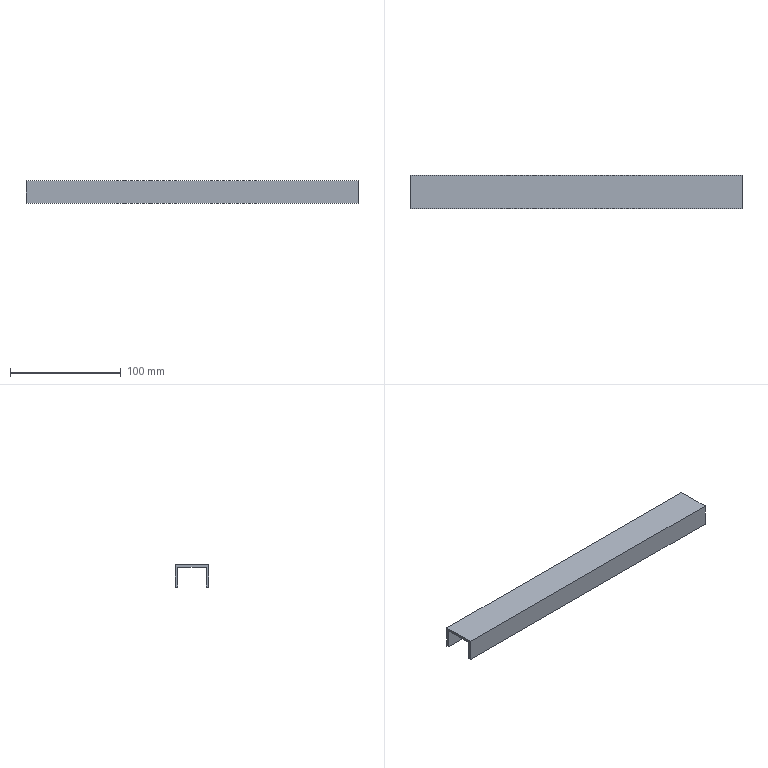Component | SolidWorks | Copy_of_Copy_of_Part3-1 | 1 solid | 10 faces | box 300 x 30 x 20 mm | volume 39600 mm3 | plane 10
build123d program:
from build123d import *

# Parameters (mm, degrees)
EXTRUDE_THIN1_DEPTH = 300


with BuildPart() as part:
    # Sketch1 → Extrude-Thin1 (new body)
    with BuildSketch(Plane.XY):
        Polygon((-20, 15.876), (0, 15.876), (0, -14.124), (-20, -14.124), (-20, -12.124), (-2, -12.124), (-2, 13.876), (-20, 13.876), align=None)
    extrude(amount=EXTRUDE_THIN1_DEPTH)


solid = part.part

# Placed as in the assembly
solid = solid.moved(Location((150, 414.124, -316.092), (0, -90, 0)))
STEP:
#1=COLOUR_RGB('',0.7922,0.8196,0.9333);
#2=FILL_AREA_STYLE_COLOUR('',#1);
#3=FILL_AREA_STYLE('',(#2));
#4=SURFACE_STYLE_FILL_AREA(#3);
#5=SURFACE_SIDE_STYLE('',(#4));
#6=SURFACE_STYLE_USAGE(.BOTH.,#5);
#7=PRESENTATION_STYLE_ASSIGNMENT((#6));
#8=CARTESIAN_POINT('',(5.906,15.827,-12.523));
#9=VERTEX_POINT('',#8);
#10=CARTESIAN_POINT('',(5.906,15.827,-13.232));
#11=VERTEX_POINT('',#10);
#12=CARTESIAN_POINT('',(5.906,15.827,-12.445));
#13=DIRECTION('',(-0.,-0.,-1.));
#14=VECTOR('',#13,39.37);
#15=LINE('',#12,#14);
#16=EDGE_CURVE('',#9,#11,#15,.T.);
#17=ORIENTED_EDGE('',*,*,#16,.T.);
#18=CARTESIAN_POINT('',(-5.906,15.827,-13.232));
#19=VERTEX_POINT('',#18);
#20=CARTESIAN_POINT('',(-5.906,15.827,-13.232));
#21=DIRECTION('',(1.,0.,-0.));
#22=VECTOR('',#21,39.37);
#23=LINE('',#20,#22);
#24=EDGE_CURVE('',#19,#11,#23,.T.);
#25=ORIENTED_EDGE('',*,*,#24,.F.);
#26=CARTESIAN_POINT('',(-5.906,15.827,-12.523));
#27=VERTEX_POINT('',#26);
#28=CARTESIAN_POINT('',(-5.906,15.827,-12.445));
#29=DIRECTION('',(-0.,-0.,-1.));
#30=VECTOR('',#29,39.37);
#31=LINE('',#28,#30);
#32=EDGE_CURVE('',#27,#19,#31,.T.);
#33=ORIENTED_EDGE('',*,*,#32,.F.);
#34=CARTESIAN_POINT('',(-5.906,15.827,-12.523));
#35=DIRECTION('',(1.,0.,-0.));
#36=VECTOR('',#35,39.37);
#37=LINE('',#34,#36);
#38=EDGE_CURVE('',#27,#9,#37,.T.);
#39=ORIENTED_EDGE('',*,*,#38,.T.);
#40=EDGE_LOOP('',(#17,#25,#33,#39));
#41=FACE_OUTER_BOUND('',#40,.T.);
#42=CARTESIAN_POINT('',(-5.906,15.827,-12.445));
#43=DIRECTION('',(0.,-1.,0.));
#44=DIRECTION('',(0.,0.,1.));
#45=AXIS2_PLACEMENT_3D('',#42,#43,#44);
#46=PLANE('',#45);
#47=ADVANCED_FACE('',(#41),#46,.F.);
#48=CARTESIAN_POINT('',(5.906,15.748,-13.232));
#49=VERTEX_POINT('',#48);
#50=CARTESIAN_POINT('',(5.906,15.748,-13.232));
#51=DIRECTION('',(-0.,1.,-0.));
#52=VECTOR('',#51,39.37);
#53=LINE('',#50,#52);
#54=EDGE_CURVE('',#49,#11,#53,.T.);
#55=ORIENTED_EDGE('',*,*,#54,.F.);
#56=CARTESIAN_POINT('',(-5.906,15.748,-13.232));
#57=VERTEX_POINT('',#56);
#58=CARTESIAN_POINT('',(-5.906,15.748,-13.232));
#59=DIRECTION('',(1.,0.,-0.));
#60=VECTOR('',#59,39.37);
#61=LINE('',#58,#60);
#62=EDGE_CURVE('',#57,#49,#61,.T.);
#63=ORIENTED_EDGE('',*,*,#62,.F.);
#64=CARTESIAN_POINT('',(-5.906,15.748,-13.232));
#65=DIRECTION('',(-0.,1.,-0.));
#66=VECTOR('',#65,39.37);
#67=LINE('',#64,#66);
#68=EDGE_CURVE('',#57,#19,#67,.T.);
#69=ORIENTED_EDGE('',*,*,#68,.T.);
#70=ORIENTED_EDGE('',*,*,#24,.T.);
#71=EDGE_LOOP('',(#55,#63,#69,#70));
#72=FACE_OUTER_BOUND('',#71,.T.);
#73=CARTESIAN_POINT('',(-5.906,15.748,-13.232));
#74=DIRECTION('',(-0.,-0.,-1.));
#75=DIRECTION('',(-1.,-0.,0.));
#76=AXIS2_PLACEMENT_3D('',#73,#74,#75);
#77=PLANE('',#76);
#78=ADVANCED_FACE('',(#72),#77,.T.);
#79=CARTESIAN_POINT('',(5.906,15.748,-12.445));
#80=VERTEX_POINT('',#79);
#81=CARTESIAN_POINT('',(5.906,15.748,-12.445));
#82=DIRECTION('',(-0.,-0.,-1.));
#83=VECTOR('',#82,39.37);
#84=LINE('',#81,#83);
#85=EDGE_CURVE('',#80,#49,#84,.T.);
#86=ORIENTED_EDGE('',*,*,#85,.F.);
#87=CARTESIAN_POINT('',(-5.906,15.748,-12.445));
#88=VERTEX_POINT('',#87);
#89=CARTESIAN_POINT('',(-5.906,15.748,-12.445));
#90=DIRECTION('',(1.,0.,-0.));
#91=VECTOR('',#90,39.37);
#92=LINE('',#89,#91);
#93=EDGE_CURVE('',#88,#80,#92,.T.);
#94=ORIENTED_EDGE('',*,*,#93,.F.);
#95=CARTESIAN_POINT('',(-5.906,15.748,-12.445));
#96=DIRECTION('',(-0.,-0.,-1.));
#97=VECTOR('',#96,39.37);
#98=LINE('',#95,#97);
#99=EDGE_CURVE('',#88,#57,#98,.T.);
#100=ORIENTED_EDGE('',*,*,#99,.T.);
#101=ORIENTED_EDGE('',*,*,#62,.T.);
#102=EDGE_LOOP('',(#86,#94,#100,#101));
#103=FACE_OUTER_BOUND('',#102,.T.);
#104=CARTESIAN_POINT('',(-5.906,15.748,-12.445));
#105=DIRECTION('',(0.,-1.,0.));
#106=DIRECTION('',(0.,0.,1.));
#107=AXIS2_PLACEMENT_3D('',#104,#105,#106);
#108=PLANE('',#107);
#109=ADVANCED_FACE('',(#103),#108,.T.);
#110=CARTESIAN_POINT('',(5.906,16.929,-12.445));
#111=VERTEX_POINT('',#110);
#112=CARTESIAN_POINT('',(5.906,15.748,-12.445));
#113=DIRECTION('',(0.,-1.,0.));
#114=VECTOR('',#113,39.37);
#115=LINE('',#112,#114);
#116=EDGE_CURVE('',#111,#80,#115,.T.);
#117=ORIENTED_EDGE('',*,*,#116,.F.);
#118=CARTESIAN_POINT('',(-5.906,16.929,-12.445));
#119=VERTEX_POINT('',#118);
#120=CARTESIAN_POINT('',(-5.906,16.929,-12.445));
#121=DIRECTION('',(1.,0.,-0.));
#122=VECTOR('',#121,39.37);
#123=LINE('',#120,#122);
#124=EDGE_CURVE('',#119,#111,#123,.T.);
#125=ORIENTED_EDGE('',*,*,#124,.F.);
#126=CARTESIAN_POINT('',(-5.906,15.748,-12.445));
#127=DIRECTION('',(0.,-1.,0.));
#128=VECTOR('',#127,39.37);
#129=LINE('',#126,#128);
#130=EDGE_CURVE('',#119,#88,#129,.T.);
#131=ORIENTED_EDGE('',*,*,#130,.T.);
#132=ORIENTED_EDGE('',*,*,#93,.T.);
#133=EDGE_LOOP('',(#117,#125,#131,#132));
#134=FACE_OUTER_BOUND('',#133,.T.);
#135=CARTESIAN_POINT('',(-5.906,15.748,-12.445));
#136=DIRECTION('',(0.,0.,1.));
#137=DIRECTION('',(1.,0.,-0.));
#138=AXIS2_PLACEMENT_3D('',#135,#136,#137);
#139=PLANE('',#138);
#140=ADVANCED_FACE('',(#134),#139,.T.);
#141=CARTESIAN_POINT('',(5.906,16.929,-13.232));
#142=VERTEX_POINT('',#141);
#143=CARTESIAN_POINT('',(5.906,16.929,-12.445));
#144=DIRECTION('',(0.,0.,1.));
#145=VECTOR('',#144,39.37);
#146=LINE('',#143,#145);
#147=EDGE_CURVE('',#142,#111,#146,.T.);
#148=ORIENTED_EDGE('',*,*,#147,.F.);
#149=CARTESIAN_POINT('',(-5.906,16.929,-13.232));
#150=VERTEX_POINT('',#149);
#151=CARTESIAN_POINT('',(-5.906,16.929,-13.232));
#152=DIRECTION('',(1.,0.,-0.));
#153=VECTOR('',#152,39.37);
#154=LINE('',#151,#153);
#155=EDGE_CURVE('',#150,#142,#154,.T.);
#156=ORIENTED_EDGE('',*,*,#155,.F.);
#157=CARTESIAN_POINT('',(-5.906,16.929,-12.445));
#158=DIRECTION('',(0.,0.,1.));
#159=VECTOR('',#158,39.37);
#160=LINE('',#157,#159);
#161=EDGE_CURVE('',#150,#119,#160,.T.);
#162=ORIENTED_EDGE('',*,*,#161,.T.);
#163=ORIENTED_EDGE('',*,*,#124,.T.);
#164=EDGE_LOOP('',(#148,#156,#162,#163));
#165=FACE_OUTER_BOUND('',#164,.T.);
#166=CARTESIAN_POINT('',(-5.906,16.929,-12.445));
#167=DIRECTION('',(-0.,1.,-0.));
#168=DIRECTION('',(-1.,-0.,0.));
#169=AXIS2_PLACEMENT_3D('',#166,#167,#168);
#170=PLANE('',#169);
#171=ADVANCED_FACE('',(#165),#170,.T.);
#172=CARTESIAN_POINT('',(5.906,16.85,-13.232));
#173=VERTEX_POINT('',#172);
#174=CARTESIAN_POINT('',(5.906,16.85,-13.232));
#175=DIRECTION('',(-0.,1.,-0.));
#176=VECTOR('',#175,39.37);
#177=LINE('',#174,#176);
#178=EDGE_CURVE('',#173,#142,#177,.T.);
#179=ORIENTED_EDGE('',*,*,#178,.F.);
#180=CARTESIAN_POINT('',(-5.906,16.85,-13.232));
#181=VERTEX_POINT('',#180);
#182=CARTESIAN_POINT('',(-5.906,16.85,-13.232));
#183=DIRECTION('',(1.,0.,-0.));
#184=VECTOR('',#183,39.37);
#185=LINE('',#182,#184);
#186=EDGE_CURVE('',#181,#173,#185,.T.);
#187=ORIENTED_EDGE('',*,*,#186,.F.);
#188=CARTESIAN_POINT('',(-5.906,16.85,-13.232));
#189=DIRECTION('',(-0.,1.,-0.));
#190=VECTOR('',#189,39.37);
#191=LINE('',#188,#190);
#192=EDGE_CURVE('',#181,#150,#191,.T.);
#193=ORIENTED_EDGE('',*,*,#192,.T.);
#194=ORIENTED_EDGE('',*,*,#155,.T.);
#195=EDGE_LOOP('',(#179,#187,#193,#194));
#196=FACE_OUTER_BOUND('',#195,.T.);
#197=CARTESIAN_POINT('',(-5.906,16.85,-13.232));
#198=DIRECTION('',(-0.,-0.,-1.));
#199=DIRECTION('',(-1.,-0.,0.));
#200=AXIS2_PLACEMENT_3D('',#197,#198,#199);
#201=PLANE('',#200);
#202=ADVANCED_FACE('',(#196),#201,.T.);
#203=CARTESIAN_POINT('',(5.906,16.85,-12.523));
#204=VERTEX_POINT('',#203);
#205=CARTESIAN_POINT('',(5.906,16.85,-12.445));
#206=DIRECTION('',(0.,0.,1.));
#207=VECTOR('',#206,39.37);
#208=LINE('',#205,#207);
#209=EDGE_CURVE('',#173,#204,#208,.T.);
#210=ORIENTED_EDGE('',*,*,#209,.T.);
#211=CARTESIAN_POINT('',(-5.906,16.85,-12.523));
#212=VERTEX_POINT('',#211);
#213=CARTESIAN_POINT('',(-5.906,16.85,-12.523));
#214=DIRECTION('',(1.,0.,-0.));
#215=VECTOR('',#214,39.37);
#216=LINE('',#213,#215);
#217=EDGE_CURVE('',#212,#204,#216,.T.);
#218=ORIENTED_EDGE('',*,*,#217,.F.);
#219=CARTESIAN_POINT('',(-5.906,16.85,-12.445));
#220=DIRECTION('',(0.,0.,1.));
#221=VECTOR('',#220,39.37);
#222=LINE('',#219,#221);
#223=EDGE_CURVE('',#181,#212,#222,.T.);
#224=ORIENTED_EDGE('',*,*,#223,.F.);
#225=ORIENTED_EDGE('',*,*,#186,.T.);
#226=EDGE_LOOP('',(#210,#218,#224,#225));
#227=FACE_OUTER_BOUND('',#226,.T.);
#228=CARTESIAN_POINT('',(-5.906,16.85,-12.445));
#229=DIRECTION('',(-0.,1.,-0.));
#230=DIRECTION('',(-1.,-0.,0.));
#231=AXIS2_PLACEMENT_3D('',#228,#229,#230);
#232=PLANE('',#231);
#233=ADVANCED_FACE('',(#227),#232,.F.);
#234=CARTESIAN_POINT('',(5.906,15.748,-12.523));
#235=DIRECTION('',(0.,-1.,0.));
#236=VECTOR('',#235,39.37);
#237=LINE('',#234,#236);
#238=EDGE_CURVE('',#204,#9,#237,.T.);
#239=ORIENTED_EDGE('',*,*,#238,.T.);
#240=ORIENTED_EDGE('',*,*,#38,.F.);
#241=CARTESIAN_POINT('',(-5.906,15.748,-12.523));
#242=DIRECTION('',(0.,-1.,0.));
#243=VECTOR('',#242,39.37);
#244=LINE('',#241,#243);
#245=EDGE_CURVE('',#212,#27,#244,.T.);
#246=ORIENTED_EDGE('',*,*,#245,.F.);
#247=ORIENTED_EDGE('',*,*,#217,.T.);
#248=EDGE_LOOP('',(#239,#240,#246,#247));
#249=FACE_OUTER_BOUND('',#248,.T.);
#250=CARTESIAN_POINT('',(-5.906,15.748,-12.523));
#251=DIRECTION('',(0.,0.,1.));
#252=DIRECTION('',(1.,0.,-0.));
#253=AXIS2_PLACEMENT_3D('',#250,#251,#252);
#254=PLANE('',#253);
#255=ADVANCED_FACE('',(#249),#254,.F.);
#256=ORIENTED_EDGE('',*,*,#32,.T.);
#257=ORIENTED_EDGE('',*,*,#68,.F.);
#258=ORIENTED_EDGE('',*,*,#99,.F.);
#259=ORIENTED_EDGE('',*,*,#130,.F.);
#260=ORIENTED_EDGE('',*,*,#161,.F.);
#261=ORIENTED_EDGE('',*,*,#192,.F.);
#262=ORIENTED_EDGE('',*,*,#223,.T.);
#263=ORIENTED_EDGE('',*,*,#245,.T.);
#264=EDGE_LOOP('',(#256,#257,#258,#259,#260,#261,#262,#263));
#265=FACE_OUTER_BOUND('',#264,.T.);
#266=CARTESIAN_POINT('',(-5.906,16.304,-12.445));
#267=DIRECTION('',(1.,0.,-0.));
#268=DIRECTION('',(-0.,-0.,-1.));
#269=AXIS2_PLACEMENT_3D('',#266,#267,#268);
#270=PLANE('',#269);
#271=ADVANCED_FACE('',(#265),#270,.F.);
#272=ORIENTED_EDGE('',*,*,#16,.F.);
#273=ORIENTED_EDGE('',*,*,#238,.F.);
#274=ORIENTED_EDGE('',*,*,#209,.F.);
#275=ORIENTED_EDGE('',*,*,#178,.T.);
#276=ORIENTED_EDGE('',*,*,#147,.T.);
#277=ORIENTED_EDGE('',*,*,#116,.T.);
#278=ORIENTED_EDGE('',*,*,#85,.T.);
#279=ORIENTED_EDGE('',*,*,#54,.T.);
#280=EDGE_LOOP('',(#272,#273,#274,#275,#276,#277,#278,#279));
#281=FACE_OUTER_BOUND('',#280,.T.);
#282=CARTESIAN_POINT('',(5.906,16.304,-12.445));
#283=DIRECTION('',(1.,0.,-0.));
#284=DIRECTION('',(-0.,-0.,-1.));
#285=AXIS2_PLACEMENT_3D('',#282,#283,#284);
#286=PLANE('',#285);
#287=ADVANCED_FACE('',(#281),#286,.T.);
#288=CLOSED_SHELL('',(#47,#78,#109,#140,#171,#202,#233,#255,#271,#287));
#289=MANIFOLD_SOLID_BREP('',#288);
#290=STYLED_ITEM('',(#7),#289);
#291=PRESENTATION_LAYER_ASSIGNMENT('','',(#290));
#292=CARTESIAN_POINT('',(0.,0.,0.));
#293=DIRECTION('',(0.,0.,1.));
#294=DIRECTION('',(1.,0.,0.));
#295=AXIS2_PLACEMENT_3D('',#292,#293,#294);
#296=(LENGTH_UNIT()NAMED_UNIT(*)SI_UNIT($,.METRE.));
#297=LENGTH_MEASURE_WITH_UNIT(LENGTH_MEASURE(0.0254),#296);
#298=DIMENSIONAL_EXPONENTS(1.,0.,0.,0.,0.,0.,0.);
#299=(CONVERSION_BASED_UNIT('',#297)LENGTH_UNIT()NAMED_UNIT(#298));
#300=UNCERTAINTY_MEASURE_WITH_UNIT(LENGTH_MEASURE(0.00001),#299,'','');
#301=(NAMED_UNIT(*)PLANE_ANGLE_UNIT()SI_UNIT($,.RADIAN.));
#302=(NAMED_UNIT(*)SI_UNIT($,.STERADIAN.)SOLID_ANGLE_UNIT());
#303=(GEOMETRIC_REPRESENTATION_CONTEXT(3)GLOBAL_UNCERTAINTY_ASSIGNED_CONTEXT((#300))GLOBAL_UNIT_ASSIGNED_CONTEXT((#299,#301,#302))REPRESENTATION_CONTEXT('',''));
#304=ADVANCED_BREP_SHAPE_REPRESENTATION('',(#289,#295),#303);
#305=(LENGTH_UNIT()NAMED_UNIT(*)SI_UNIT($,.METRE.));
#306=LENGTH_MEASURE_WITH_UNIT(LENGTH_MEASURE(0.0254),#305);
#307=DIMENSIONAL_EXPONENTS(1.,0.,0.,0.,0.,0.,0.);
#308=(CONVERSION_BASED_UNIT('',#306)LENGTH_UNIT()NAMED_UNIT(#307));
#309=UNCERTAINTY_MEASURE_WITH_UNIT(LENGTH_MEASURE(0.00001),#308,'','');
#310=(NAMED_UNIT(*)PLANE_ANGLE_UNIT()SI_UNIT($,.RADIAN.));
#311=(NAMED_UNIT(*)SI_UNIT($,.STERADIAN.)SOLID_ANGLE_UNIT());
#312=(GEOMETRIC_REPRESENTATION_CONTEXT(3)GLOBAL_UNCERTAINTY_ASSIGNED_CONTEXT((#309))GLOBAL_UNIT_ASSIGNED_CONTEXT((#308,#310,#311))REPRESENTATION_CONTEXT('',''));
#313=MECHANICAL_DESIGN_GEOMETRIC_PRESENTATION_REPRESENTATION('',(#290),#312);